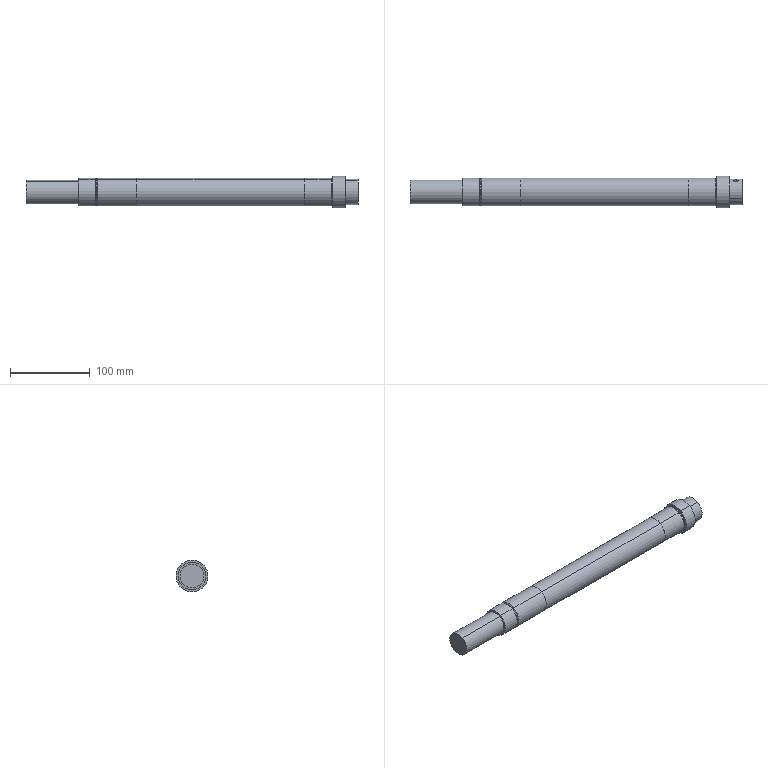Component | SolidWorks | 2-10-10WorkpieceAxisAssembly-1_2-10-2WorkpieceAxis-1 | 1 solid | 40 faces | volume 381179 mm3 | cylinder 24 | plane 12 | cone 4 | commonest cylinder face diameters 35 x6 32 x4 30 x2 6 x2 6.8 x2 20 x2 34.8 x2 34 x2